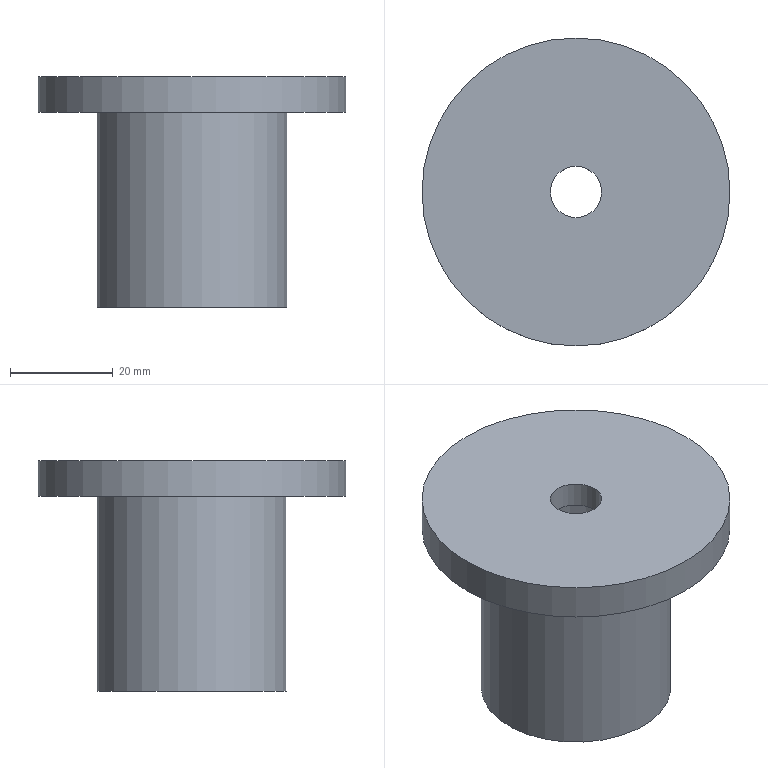Component | NX | SHAFT_SLEEVE | 1 solid | 8 faces | box 60 x 60 x 45 mm | volume 37355 mm3 | cylinder 4 | plane 4 | commonest cylinder face diameters 10 x1 27 x1 37 x1 60 x1
STEP:
#1=CARTESIAN_POINT('',(0.,0.,0.));
#2=DIRECTION('',(0.,0.,1.));
#3=DIRECTION('',(1.,0.,0.));
#4=AXIS2_PLACEMENT_3D('',#1,#2,#3);
#5=CARTESIAN_POINT('',(-146.777,5.,111.491));
#6=VERTEX_POINT('',#5);
#7=CARTESIAN_POINT('',(-146.777,0.,111.491));
#8=DIRECTION('',(0.,0.,-1.));
#9=DIRECTION('',(0.,1.,0.));
#10=AXIS2_PLACEMENT_3D('',#7,#8,#9);
#11=CIRCLE('',#10,5.);
#12=CARTESIAN_POINT('',(-146.777,0.,109.491));
#13=DIRECTION('',(0.,0.,-1.));
#14=DIRECTION('',(0.,1.,0.));
#15=AXIS2_PLACEMENT_3D('',#12,#13,#14);
#16=CYLINDRICAL_SURFACE('',#15,5.);
#17=CARTESIAN_POINT('',(0.,-2.));
#18=DIRECTION('',(1.,0.));
#19=VECTOR('',#18,1.);
#20=LINE('',#17,#19);
#21=(GEOMETRIC_REPRESENTATION_CONTEXT(2)PARAMETRIC_REPRESENTATION_CONTEXT()REPRESENTATION_CONTEXT('',''));
#22=DEFINITIONAL_REPRESENTATION('',(#20),#21);
#23=PCURVE('',#16,#22);
#24=CARTESIAN_POINT('',(-141.777,0.,111.491));
#25=DIRECTION('',(0.,0.,-1.));
#26=DIRECTION('',(0.,1.,0.));
#27=AXIS2_PLACEMENT_3D('',#24,#25,#26);
#28=PLANE('',#27);
#29=CARTESIAN_POINT('',(0.,-5.));
#30=DIRECTION('',(1.,0.));
#31=AXIS2_PLACEMENT_2D('',#29,#30);
#32=CIRCLE('',#31,5.);
#33=(GEOMETRIC_REPRESENTATION_CONTEXT(2)PARAMETRIC_REPRESENTATION_CONTEXT()REPRESENTATION_CONTEXT('',''));
#34=DEFINITIONAL_REPRESENTATION('',(#32),#33);
#35=PCURVE('',#28,#34);
#36=SURFACE_CURVE('',#11,(#23,#35),.PCURVE_S1.);
#37=EDGE_CURVE('',#6,#6,#36,.T.);
#38=ORIENTED_EDGE('',*,*,#37,.F.);
#39=CARTESIAN_POINT('',(-146.777,5.,116.491));
#40=VERTEX_POINT('',#39);
#41=CARTESIAN_POINT('',(-146.777,5.,116.491));
#42=CARTESIAN_POINT('',(-146.777,5.,111.491));
#43=B_SPLINE_CURVE_WITH_KNOTS('',1,(#41,#42),.UNSPECIFIED.,.F.,.F.,(2,2),(-7.,-2.),.PIECEWISE_BEZIER_KNOTS.);
#44=CARTESIAN_POINT('',(0.,0.));
#45=DIRECTION('',(0.,1.));
#46=VECTOR('',#45,1.);
#47=LINE('',#44,#46);
#48=(GEOMETRIC_REPRESENTATION_CONTEXT(2)PARAMETRIC_REPRESENTATION_CONTEXT()REPRESENTATION_CONTEXT('',''));
#49=DEFINITIONAL_REPRESENTATION('',(#47),#48);
#50=PCURVE('',#16,#49);
#51=CARTESIAN_POINT('',(6.283,0.));
#52=DIRECTION('',(0.,1.));
#53=VECTOR('',#52,1.);
#54=LINE('',#51,#53);
#55=(GEOMETRIC_REPRESENTATION_CONTEXT(2)PARAMETRIC_REPRESENTATION_CONTEXT()REPRESENTATION_CONTEXT('',''));
#56=DEFINITIONAL_REPRESENTATION('',(#54),#55);
#57=PCURVE('',#16,#56);
#58=SEAM_CURVE('',#43,(#50,#57),.PCURVE_S1.);
#59=EDGE_CURVE('',#40,#6,#58,.T.);
#60=ORIENTED_EDGE('',*,*,#59,.F.);
#61=CARTESIAN_POINT('',(-146.777,0.,116.491));
#62=DIRECTION('',(0.,0.,-1.));
#63=DIRECTION('',(0.,1.,0.));
#64=AXIS2_PLACEMENT_3D('',#61,#62,#63);
#65=CIRCLE('',#64,5.);
#66=CARTESIAN_POINT('',(0.,-7.));
#67=DIRECTION('',(1.,0.));
#68=VECTOR('',#67,1.);
#69=LINE('',#66,#68);
#70=(GEOMETRIC_REPRESENTATION_CONTEXT(2)PARAMETRIC_REPRESENTATION_CONTEXT()REPRESENTATION_CONTEXT('',''));
#71=DEFINITIONAL_REPRESENTATION('',(#69),#70);
#72=PCURVE('',#16,#71);
#73=CARTESIAN_POINT('',(-116.777,0.,116.491));
#74=DIRECTION('',(0.,0.,1.));
#75=DIRECTION('',(0.,-1.,0.));
#76=AXIS2_PLACEMENT_3D('',#73,#74,#75);
#77=PLANE('',#76);
#78=CARTESIAN_POINT('',(-5.,-30.));
#79=CARTESIAN_POINT('',(-5.,-21.34));
#80=CARTESIAN_POINT('',(2.5,-25.67));
#81=CARTESIAN_POINT('',(10.,-30.));
#82=CARTESIAN_POINT('',(2.5,-34.33));
#83=CARTESIAN_POINT('',(-5.,-38.66));
#84=CARTESIAN_POINT('',(-5.,-30.));
#85=(BOUNDED_CURVE()B_SPLINE_CURVE(2,(#78,#79,#80,#81,#82,#83,#84),.UNSPECIFIED.,.T.,.F.)B_SPLINE_CURVE_WITH_KNOTS((1,2,2,2,2,1),(-2.094,0.,2.094,4.189,6.283,8.378),.UNSPECIFIED.)CURVE()GEOMETRIC_REPRESENTATION_ITEM()RATIONAL_B_SPLINE_CURVE((1.,0.5,1.,0.5,1.,0.5,1.))REPRESENTATION_ITEM(''));
#86=(GEOMETRIC_REPRESENTATION_CONTEXT(2)PARAMETRIC_REPRESENTATION_CONTEXT()REPRESENTATION_CONTEXT('',''));
#87=DEFINITIONAL_REPRESENTATION('',(#85),#86);
#88=PCURVE('',#77,#87);
#89=SURFACE_CURVE('',#65,(#72,#88),.PCURVE_S1.);
#90=EDGE_CURVE('',#40,#40,#89,.T.);
#91=ORIENTED_EDGE('',*,*,#90,.T.);
#92=ORIENTED_EDGE('',*,*,#59,.T.);
#93=EDGE_LOOP('',(#38,#60,#91,#92));
#94=FACE_BOUND('',#93,.F.);
#95=ADVANCED_FACE('',(#94),#16,.F.);
#96=CARTESIAN_POINT('',(-146.777,13.5,111.491));
#97=VERTEX_POINT('',#96);
#98=CARTESIAN_POINT('',(-146.777,0.,111.491));
#99=DIRECTION('',(0.,0.,-1.));
#100=DIRECTION('',(0.,1.,0.));
#101=AXIS2_PLACEMENT_3D('',#98,#99,#100);
#102=CIRCLE('',#101,13.5);
#103=CARTESIAN_POINT('',(0.,-5.));
#104=DIRECTION('',(1.,0.));
#105=AXIS2_PLACEMENT_2D('',#103,#104);
#106=CIRCLE('',#105,13.5);
#107=(GEOMETRIC_REPRESENTATION_CONTEXT(2)PARAMETRIC_REPRESENTATION_CONTEXT()REPRESENTATION_CONTEXT('',''));
#108=DEFINITIONAL_REPRESENTATION('',(#106),#107);
#109=PCURVE('',#28,#108);
#110=CARTESIAN_POINT('',(-146.777,0.,109.491));
#111=DIRECTION('',(0.,0.,-1.));
#112=DIRECTION('',(0.,1.,0.));
#113=AXIS2_PLACEMENT_3D('',#110,#111,#112);
#114=CYLINDRICAL_SURFACE('',#113,13.5);
#115=CARTESIAN_POINT('',(0.,-2.));
#116=DIRECTION('',(1.,0.));
#117=VECTOR('',#116,1.);
#118=LINE('',#115,#117);
#119=(GEOMETRIC_REPRESENTATION_CONTEXT(2)PARAMETRIC_REPRESENTATION_CONTEXT()REPRESENTATION_CONTEXT('',''));
#120=DEFINITIONAL_REPRESENTATION('',(#118),#119);
#121=PCURVE('',#114,#120);
#122=SURFACE_CURVE('',#102,(#109,#121),.PCURVE_S1.);
#123=EDGE_CURVE('',#97,#97,#122,.T.);
#124=ORIENTED_EDGE('',*,*,#123,.T.);
#125=EDGE_LOOP('',(#124));
#126=FACE_BOUND('',#125,.T.);
#127=ORIENTED_EDGE('',*,*,#37,.F.);
#128=EDGE_LOOP('',(#127));
#129=FACE_BOUND('',#128,.T.);
#130=ADVANCED_FACE('',(#126,#129),#28,.T.);
#131=CARTESIAN_POINT('',(-146.777,13.5,71.491));
#132=VERTEX_POINT('',#131);
#133=CARTESIAN_POINT('',(-146.777,0.,71.491));
#134=DIRECTION('',(0.,0.,-1.));
#135=DIRECTION('',(0.,1.,0.));
#136=AXIS2_PLACEMENT_3D('',#133,#134,#135);
#137=CIRCLE('',#136,13.5);
#138=CARTESIAN_POINT('',(0.,38.));
#139=DIRECTION('',(1.,0.));
#140=VECTOR('',#139,1.);
#141=LINE('',#138,#140);
#142=(GEOMETRIC_REPRESENTATION_CONTEXT(2)PARAMETRIC_REPRESENTATION_CONTEXT()REPRESENTATION_CONTEXT('',''));
#143=DEFINITIONAL_REPRESENTATION('',(#141),#142);
#144=PCURVE('',#114,#143);
#145=CARTESIAN_POINT('',(-133.277,0.,71.491));
#146=DIRECTION('',(0.,0.,-1.));
#147=DIRECTION('',(0.,1.,0.));
#148=AXIS2_PLACEMENT_3D('',#145,#146,#147);
#149=PLANE('',#148);
#150=CARTESIAN_POINT('',(0.,-13.5));
#151=DIRECTION('',(1.,0.));
#152=AXIS2_PLACEMENT_2D('',#150,#151);
#153=CIRCLE('',#152,13.5);
#154=(GEOMETRIC_REPRESENTATION_CONTEXT(2)PARAMETRIC_REPRESENTATION_CONTEXT()REPRESENTATION_CONTEXT('',''));
#155=DEFINITIONAL_REPRESENTATION('',(#153),#154);
#156=PCURVE('',#149,#155);
#157=SURFACE_CURVE('',#137,(#144,#156),.PCURVE_S1.);
#158=EDGE_CURVE('',#132,#132,#157,.T.);
#159=ORIENTED_EDGE('',*,*,#158,.F.);
#160=CARTESIAN_POINT('',(-146.777,13.5,111.491));
#161=CARTESIAN_POINT('',(-146.777,13.5,71.491));
#162=B_SPLINE_CURVE_WITH_KNOTS('',1,(#160,#161),.UNSPECIFIED.,.F.,.F.,(2,2),(-2.,38.),.PIECEWISE_BEZIER_KNOTS.);
#163=CARTESIAN_POINT('',(0.,0.));
#164=DIRECTION('',(0.,1.));
#165=VECTOR('',#164,1.);
#166=LINE('',#163,#165);
#167=(GEOMETRIC_REPRESENTATION_CONTEXT(2)PARAMETRIC_REPRESENTATION_CONTEXT()REPRESENTATION_CONTEXT('',''));
#168=DEFINITIONAL_REPRESENTATION('',(#166),#167);
#169=PCURVE('',#114,#168);
#170=CARTESIAN_POINT('',(6.283,0.));
#171=DIRECTION('',(0.,1.));
#172=VECTOR('',#171,1.);
#173=LINE('',#170,#172);
#174=(GEOMETRIC_REPRESENTATION_CONTEXT(2)PARAMETRIC_REPRESENTATION_CONTEXT()REPRESENTATION_CONTEXT('',''));
#175=DEFINITIONAL_REPRESENTATION('',(#173),#174);
#176=PCURVE('',#114,#175);
#177=SEAM_CURVE('',#162,(#169,#176),.PCURVE_S1.);
#178=EDGE_CURVE('',#97,#132,#177,.T.);
#179=ORIENTED_EDGE('',*,*,#178,.F.);
#180=ORIENTED_EDGE('',*,*,#123,.T.);
#181=ORIENTED_EDGE('',*,*,#178,.T.);
#182=EDGE_LOOP('',(#159,#179,#180,#181));
#183=FACE_BOUND('',#182,.F.);
#184=ADVANCED_FACE('',(#183),#114,.F.);
#185=CARTESIAN_POINT('',(-146.777,18.5,71.491));
#186=VERTEX_POINT('',#185);
#187=CARTESIAN_POINT('',(-146.777,0.,71.491));
#188=DIRECTION('',(0.,0.,-1.));
#189=DIRECTION('',(0.,1.,0.));
#190=AXIS2_PLACEMENT_3D('',#187,#188,#189);
#191=CIRCLE('',#190,18.5);
#192=CARTESIAN_POINT('',(0.,-13.5));
#193=DIRECTION('',(1.,0.));
#194=AXIS2_PLACEMENT_2D('',#192,#193);
#195=CIRCLE('',#194,18.5);
#196=(GEOMETRIC_REPRESENTATION_CONTEXT(2)PARAMETRIC_REPRESENTATION_CONTEXT()REPRESENTATION_CONTEXT('',''));
#197=DEFINITIONAL_REPRESENTATION('',(#195),#196);
#198=PCURVE('',#149,#197);
#199=CARTESIAN_POINT('',(-146.777,0.,109.491));
#200=DIRECTION('',(0.,0.,-1.));
#201=DIRECTION('',(0.,1.,0.));
#202=AXIS2_PLACEMENT_3D('',#199,#200,#201);
#203=CYLINDRICAL_SURFACE('',#202,18.5);
#204=CARTESIAN_POINT('',(0.,38.));
#205=DIRECTION('',(1.,0.));
#206=VECTOR('',#205,1.);
#207=LINE('',#204,#206);
#208=(GEOMETRIC_REPRESENTATION_CONTEXT(2)PARAMETRIC_REPRESENTATION_CONTEXT()REPRESENTATION_CONTEXT('',''));
#209=DEFINITIONAL_REPRESENTATION('',(#207),#208);
#210=PCURVE('',#203,#209);
#211=SURFACE_CURVE('',#191,(#198,#210),.PCURVE_S1.);
#212=EDGE_CURVE('',#186,#186,#211,.T.);
#213=ORIENTED_EDGE('',*,*,#212,.T.);
#214=EDGE_LOOP('',(#213));
#215=FACE_BOUND('',#214,.T.);
#216=ORIENTED_EDGE('',*,*,#158,.F.);
#217=EDGE_LOOP('',(#216));
#218=FACE_BOUND('',#217,.T.);
#219=ADVANCED_FACE('',(#215,#218),#149,.T.);
#220=CARTESIAN_POINT('',(-146.777,18.5,109.491));
#221=VERTEX_POINT('',#220);
#222=CARTESIAN_POINT('',(-146.777,0.,109.491));
#223=DIRECTION('',(0.,0.,-1.));
#224=DIRECTION('',(0.,1.,0.));
#225=AXIS2_PLACEMENT_3D('',#222,#223,#224);
#226=CIRCLE('',#225,18.5);
#227=CARTESIAN_POINT('',(0.,0.));
#228=DIRECTION('',(1.,0.));
#229=VECTOR('',#228,1.);
#230=LINE('',#227,#229);
#231=(GEOMETRIC_REPRESENTATION_CONTEXT(2)PARAMETRIC_REPRESENTATION_CONTEXT()REPRESENTATION_CONTEXT('',''));
#232=DEFINITIONAL_REPRESENTATION('',(#230),#231);
#233=PCURVE('',#203,#232);
#234=CARTESIAN_POINT('',(-128.277,0.,109.491));
#235=DIRECTION('',(0.,0.,-1.));
#236=DIRECTION('',(0.,1.,0.));
#237=AXIS2_PLACEMENT_3D('',#234,#235,#236);
#238=PLANE('',#237);
#239=CARTESIAN_POINT('',(0.,-18.5));
#240=DIRECTION('',(1.,0.));
#241=AXIS2_PLACEMENT_2D('',#239,#240);
#242=CIRCLE('',#241,18.5);
#243=(GEOMETRIC_REPRESENTATION_CONTEXT(2)PARAMETRIC_REPRESENTATION_CONTEXT()REPRESENTATION_CONTEXT('',''));
#244=DEFINITIONAL_REPRESENTATION('',(#242),#243);
#245=PCURVE('',#238,#244);
#246=SURFACE_CURVE('',#226,(#233,#245),.PCURVE_S1.);
#247=EDGE_CURVE('',#221,#221,#246,.T.);
#248=ORIENTED_EDGE('',*,*,#247,.T.);
#249=CARTESIAN_POINT('',(-146.777,18.5,109.491));
#250=CARTESIAN_POINT('',(-146.777,18.5,71.491));
#251=B_SPLINE_CURVE_WITH_KNOTS('',1,(#249,#250),.UNSPECIFIED.,.F.,.F.,(2,2),(0.,38.),.PIECEWISE_BEZIER_KNOTS.);
#252=CARTESIAN_POINT('',(6.283,0.));
#253=DIRECTION('',(0.,1.));
#254=VECTOR('',#253,1.);
#255=LINE('',#252,#254);
#256=(GEOMETRIC_REPRESENTATION_CONTEXT(2)PARAMETRIC_REPRESENTATION_CONTEXT()REPRESENTATION_CONTEXT('',''));
#257=DEFINITIONAL_REPRESENTATION('',(#255),#256);
#258=PCURVE('',#203,#257);
#259=CARTESIAN_POINT('',(0.,0.));
#260=DIRECTION('',(0.,1.));
#261=VECTOR('',#260,1.);
#262=LINE('',#259,#261);
#263=(GEOMETRIC_REPRESENTATION_CONTEXT(2)PARAMETRIC_REPRESENTATION_CONTEXT()REPRESENTATION_CONTEXT('',''));
#264=DEFINITIONAL_REPRESENTATION('',(#262),#263);
#265=PCURVE('',#203,#264);
#266=SEAM_CURVE('',#251,(#258,#265),.PCURVE_S1.);
#267=EDGE_CURVE('',#221,#186,#266,.T.);
#268=ORIENTED_EDGE('',*,*,#267,.T.);
#269=ORIENTED_EDGE('',*,*,#212,.F.);
#270=ORIENTED_EDGE('',*,*,#267,.F.);
#271=EDGE_LOOP('',(#248,#268,#269,#270));
#272=FACE_BOUND('',#271,.T.);
#273=ADVANCED_FACE('',(#272),#203,.T.);
#274=CARTESIAN_POINT('',(-146.777,30.,109.491));
#275=VERTEX_POINT('',#274);
#276=CARTESIAN_POINT('',(-146.777,0.,109.491));
#277=DIRECTION('',(0.,0.,-1.));
#278=DIRECTION('',(0.,1.,0.));
#279=AXIS2_PLACEMENT_3D('',#276,#277,#278);
#280=CIRCLE('',#279,30.);
#281=CARTESIAN_POINT('',(0.,-18.5));
#282=DIRECTION('',(1.,0.));
#283=AXIS2_PLACEMENT_2D('',#281,#282);
#284=CIRCLE('',#283,30.);
#285=(GEOMETRIC_REPRESENTATION_CONTEXT(2)PARAMETRIC_REPRESENTATION_CONTEXT()REPRESENTATION_CONTEXT('',''));
#286=DEFINITIONAL_REPRESENTATION('',(#284),#285);
#287=PCURVE('',#238,#286);
#288=CARTESIAN_POINT('',(-146.777,0.,109.491));
#289=DIRECTION('',(0.,0.,-1.));
#290=DIRECTION('',(0.,1.,0.));
#291=AXIS2_PLACEMENT_3D('',#288,#289,#290);
#292=CYLINDRICAL_SURFACE('',#291,30.);
#293=CARTESIAN_POINT('',(0.,0.));
#294=DIRECTION('',(1.,0.));
#295=VECTOR('',#294,1.);
#296=LINE('',#293,#295);
#297=(GEOMETRIC_REPRESENTATION_CONTEXT(2)PARAMETRIC_REPRESENTATION_CONTEXT()REPRESENTATION_CONTEXT('',''));
#298=DEFINITIONAL_REPRESENTATION('',(#296),#297);
#299=PCURVE('',#292,#298);
#300=SURFACE_CURVE('',#280,(#287,#299),.PCURVE_S1.);
#301=EDGE_CURVE('',#275,#275,#300,.T.);
#302=ORIENTED_EDGE('',*,*,#301,.T.);
#303=EDGE_LOOP('',(#302));
#304=FACE_BOUND('',#303,.T.);
#305=ORIENTED_EDGE('',*,*,#247,.F.);
#306=EDGE_LOOP('',(#305));
#307=FACE_BOUND('',#306,.T.);
#308=ADVANCED_FACE('',(#304,#307),#238,.T.);
#309=CARTESIAN_POINT('',(-146.777,30.,116.491));
#310=VERTEX_POINT('',#309);
#311=CARTESIAN_POINT('',(-146.777,0.,116.491));
#312=DIRECTION('',(0.,0.,-1.));
#313=DIRECTION('',(0.,1.,0.));
#314=AXIS2_PLACEMENT_3D('',#311,#312,#313);
#315=CIRCLE('',#314,30.);
#316=CARTESIAN_POINT('',(0.,-7.));
#317=DIRECTION('',(1.,0.));
#318=VECTOR('',#317,1.);
#319=LINE('',#316,#318);
#320=(GEOMETRIC_REPRESENTATION_CONTEXT(2)PARAMETRIC_REPRESENTATION_CONTEXT()REPRESENTATION_CONTEXT('',''));
#321=DEFINITIONAL_REPRESENTATION('',(#319),#320);
#322=PCURVE('',#292,#321);
#323=CARTESIAN_POINT('',(-30.,-30.));
#324=CARTESIAN_POINT('',(-30.,21.962));
#325=CARTESIAN_POINT('',(15.,-4.019));
#326=CARTESIAN_POINT('',(60.,-30.));
#327=CARTESIAN_POINT('',(15.,-55.981));
#328=CARTESIAN_POINT('',(-30.,-81.962));
#329=CARTESIAN_POINT('',(-30.,-30.));
#330=(BOUNDED_CURVE()B_SPLINE_CURVE(2,(#323,#324,#325,#326,#327,#328,#329),.UNSPECIFIED.,.T.,.F.)B_SPLINE_CURVE_WITH_KNOTS((1,2,2,2,2,1),(-2.094,0.,2.094,4.189,6.283,8.378),.UNSPECIFIED.)CURVE()GEOMETRIC_REPRESENTATION_ITEM()RATIONAL_B_SPLINE_CURVE((1.,0.5,1.,0.5,1.,0.5,1.))REPRESENTATION_ITEM(''));
#331=(GEOMETRIC_REPRESENTATION_CONTEXT(2)PARAMETRIC_REPRESENTATION_CONTEXT()REPRESENTATION_CONTEXT('',''));
#332=DEFINITIONAL_REPRESENTATION('',(#330),#331);
#333=PCURVE('',#77,#332);
#334=SURFACE_CURVE('',#315,(#322,#333),.PCURVE_S1.);
#335=EDGE_CURVE('',#310,#310,#334,.T.);
#336=ORIENTED_EDGE('',*,*,#335,.T.);
#337=CARTESIAN_POINT('',(-146.777,30.,116.491));
#338=CARTESIAN_POINT('',(-146.777,30.,109.491));
#339=B_SPLINE_CURVE_WITH_KNOTS('',1,(#337,#338),.UNSPECIFIED.,.F.,.F.,(2,2),(-7.,0.),.PIECEWISE_BEZIER_KNOTS.);
#340=CARTESIAN_POINT('',(6.283,0.));
#341=DIRECTION('',(0.,1.));
#342=VECTOR('',#341,1.);
#343=LINE('',#340,#342);
#344=(GEOMETRIC_REPRESENTATION_CONTEXT(2)PARAMETRIC_REPRESENTATION_CONTEXT()REPRESENTATION_CONTEXT('',''));
#345=DEFINITIONAL_REPRESENTATION('',(#343),#344);
#346=PCURVE('',#292,#345);
#347=CARTESIAN_POINT('',(0.,0.));
#348=DIRECTION('',(0.,1.));
#349=VECTOR('',#348,1.);
#350=LINE('',#347,#349);
#351=(GEOMETRIC_REPRESENTATION_CONTEXT(2)PARAMETRIC_REPRESENTATION_CONTEXT()REPRESENTATION_CONTEXT('',''));
#352=DEFINITIONAL_REPRESENTATION('',(#350),#351);
#353=PCURVE('',#292,#352);
#354=SEAM_CURVE('',#339,(#346,#353),.PCURVE_S1.);
#355=EDGE_CURVE('',#310,#275,#354,.T.);
#356=ORIENTED_EDGE('',*,*,#355,.T.);
#357=ORIENTED_EDGE('',*,*,#301,.F.);
#358=ORIENTED_EDGE('',*,*,#355,.F.);
#359=EDGE_LOOP('',(#336,#356,#357,#358));
#360=FACE_BOUND('',#359,.T.);
#361=ADVANCED_FACE('',(#360),#292,.T.);
#362=ORIENTED_EDGE('',*,*,#90,.T.);
#363=EDGE_LOOP('',(#362));
#364=FACE_BOUND('',#363,.T.);
#365=ORIENTED_EDGE('',*,*,#335,.F.);
#366=EDGE_LOOP('',(#365));
#367=FACE_BOUND('',#366,.T.);
#368=ADVANCED_FACE('',(#364,#367),#77,.T.);
#369=CLOSED_SHELL('',(#95,#130,#184,#219,#273,#308,#361,#368));
#370=MANIFOLD_SOLID_BREP('',#369);
#371=(LENGTH_UNIT()NAMED_UNIT(*)SI_UNIT(.MILLI.,.METRE.));
#372=UNCERTAINTY_MEASURE_WITH_UNIT(LENGTH_MEASURE(0.00001),#371,'','');
#373=(NAMED_UNIT(*)PLANE_ANGLE_UNIT()SI_UNIT($,.RADIAN.));
#374=(NAMED_UNIT(*)SI_UNIT($,.STERADIAN.)SOLID_ANGLE_UNIT());
#375=(GEOMETRIC_REPRESENTATION_CONTEXT(3)GLOBAL_UNCERTAINTY_ASSIGNED_CONTEXT((#372))GLOBAL_UNIT_ASSIGNED_CONTEXT((#371,#373,#374))REPRESENTATION_CONTEXT('',''));
#376=ADVANCED_BREP_SHAPE_REPRESENTATION('',(#4,#370),#375);